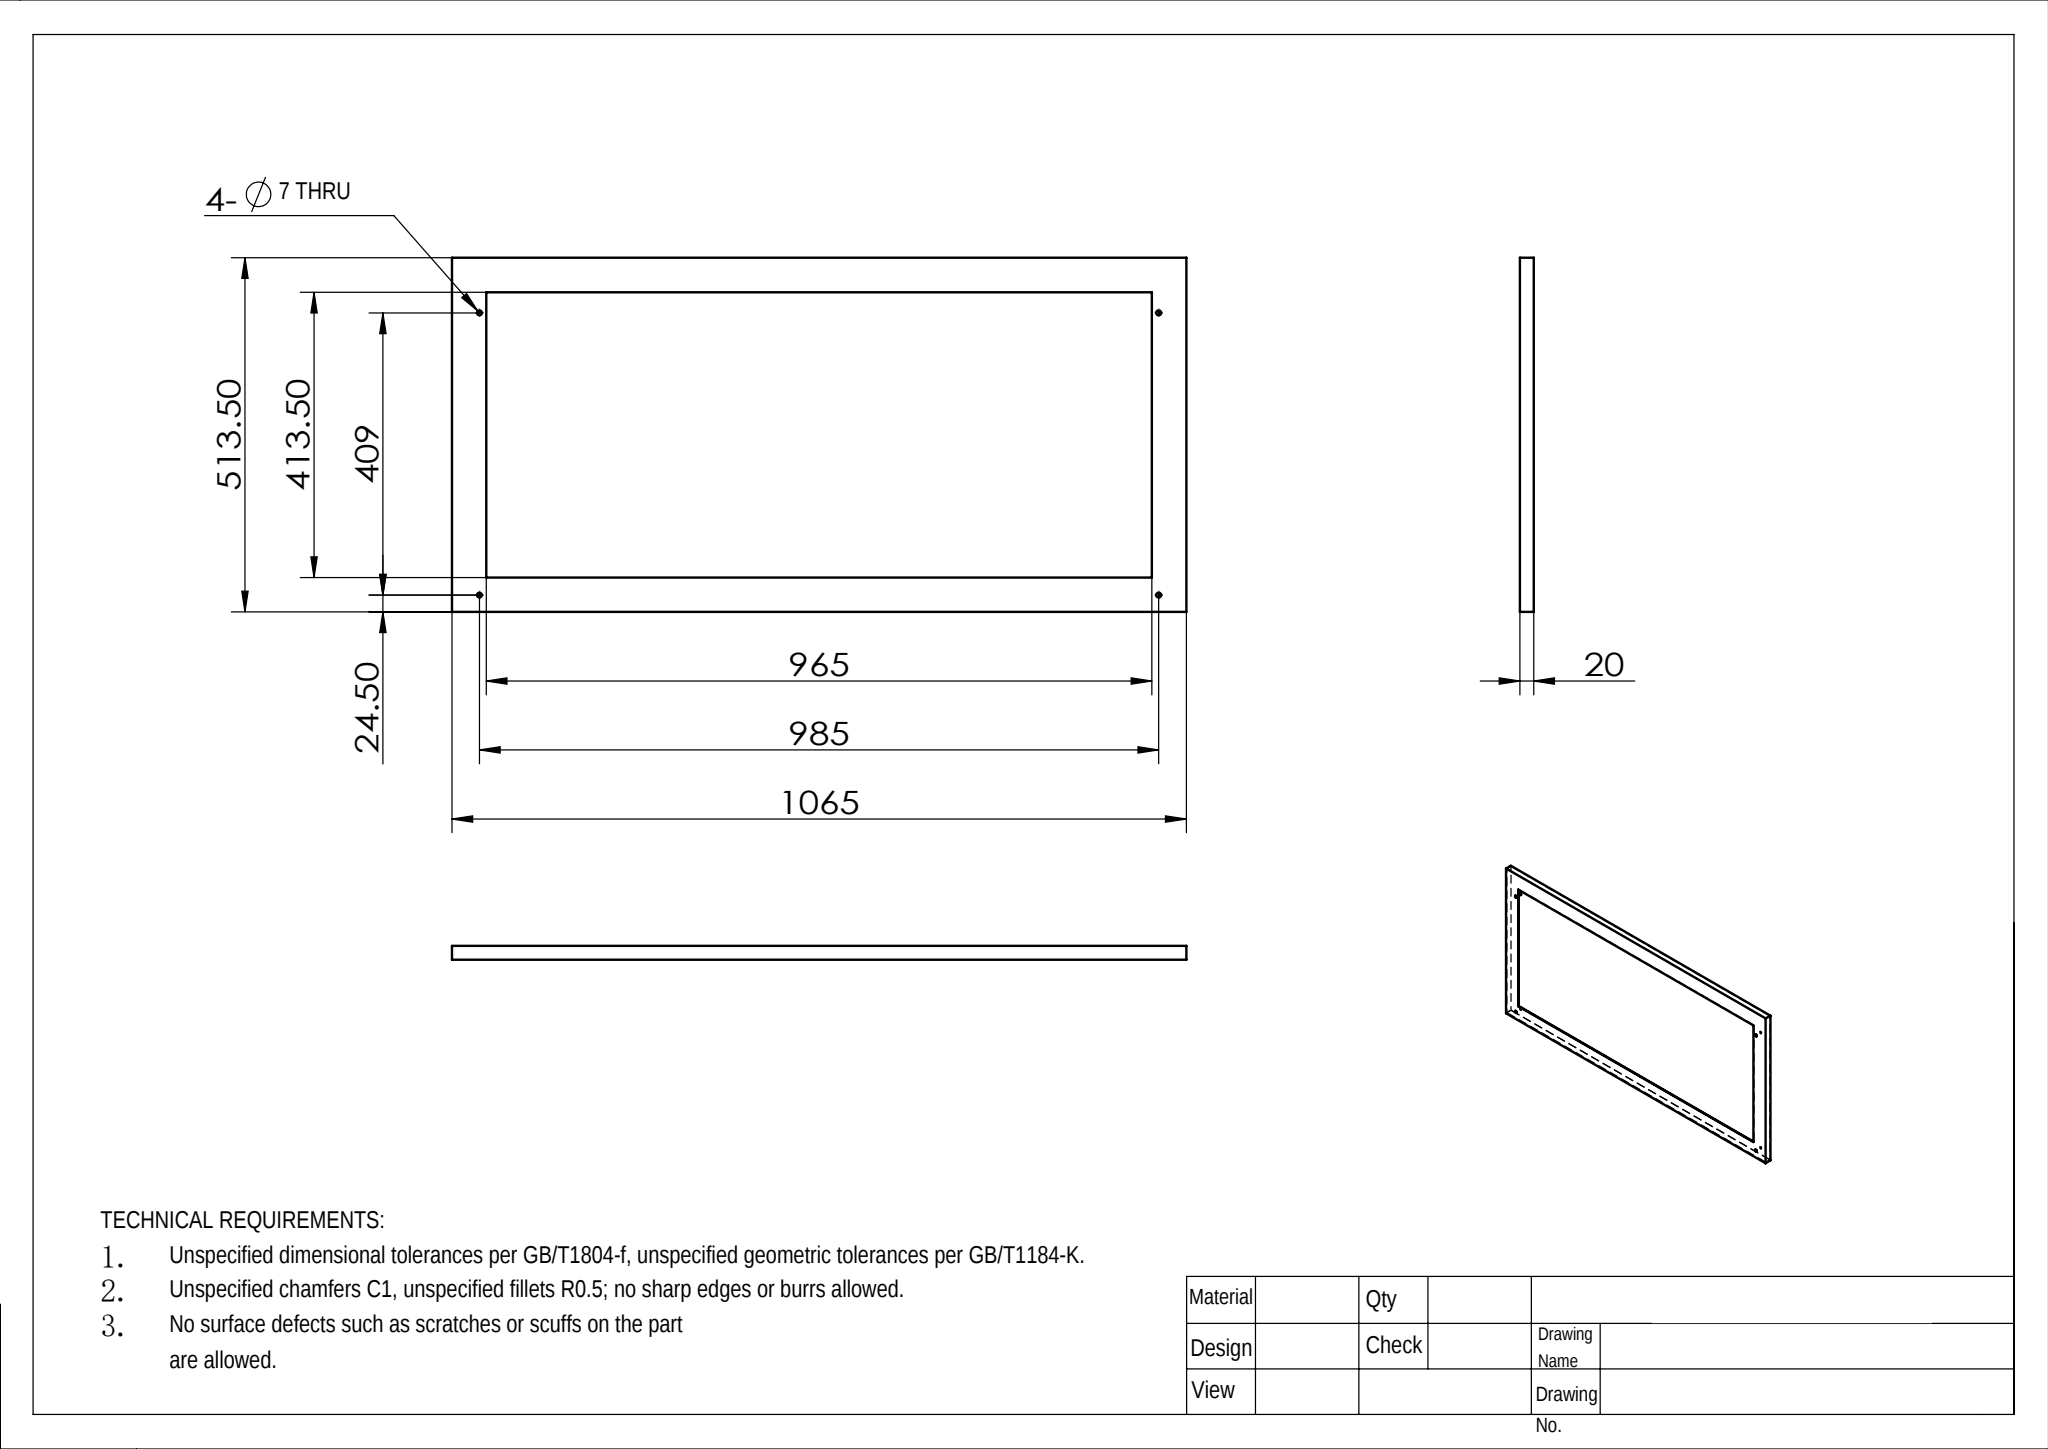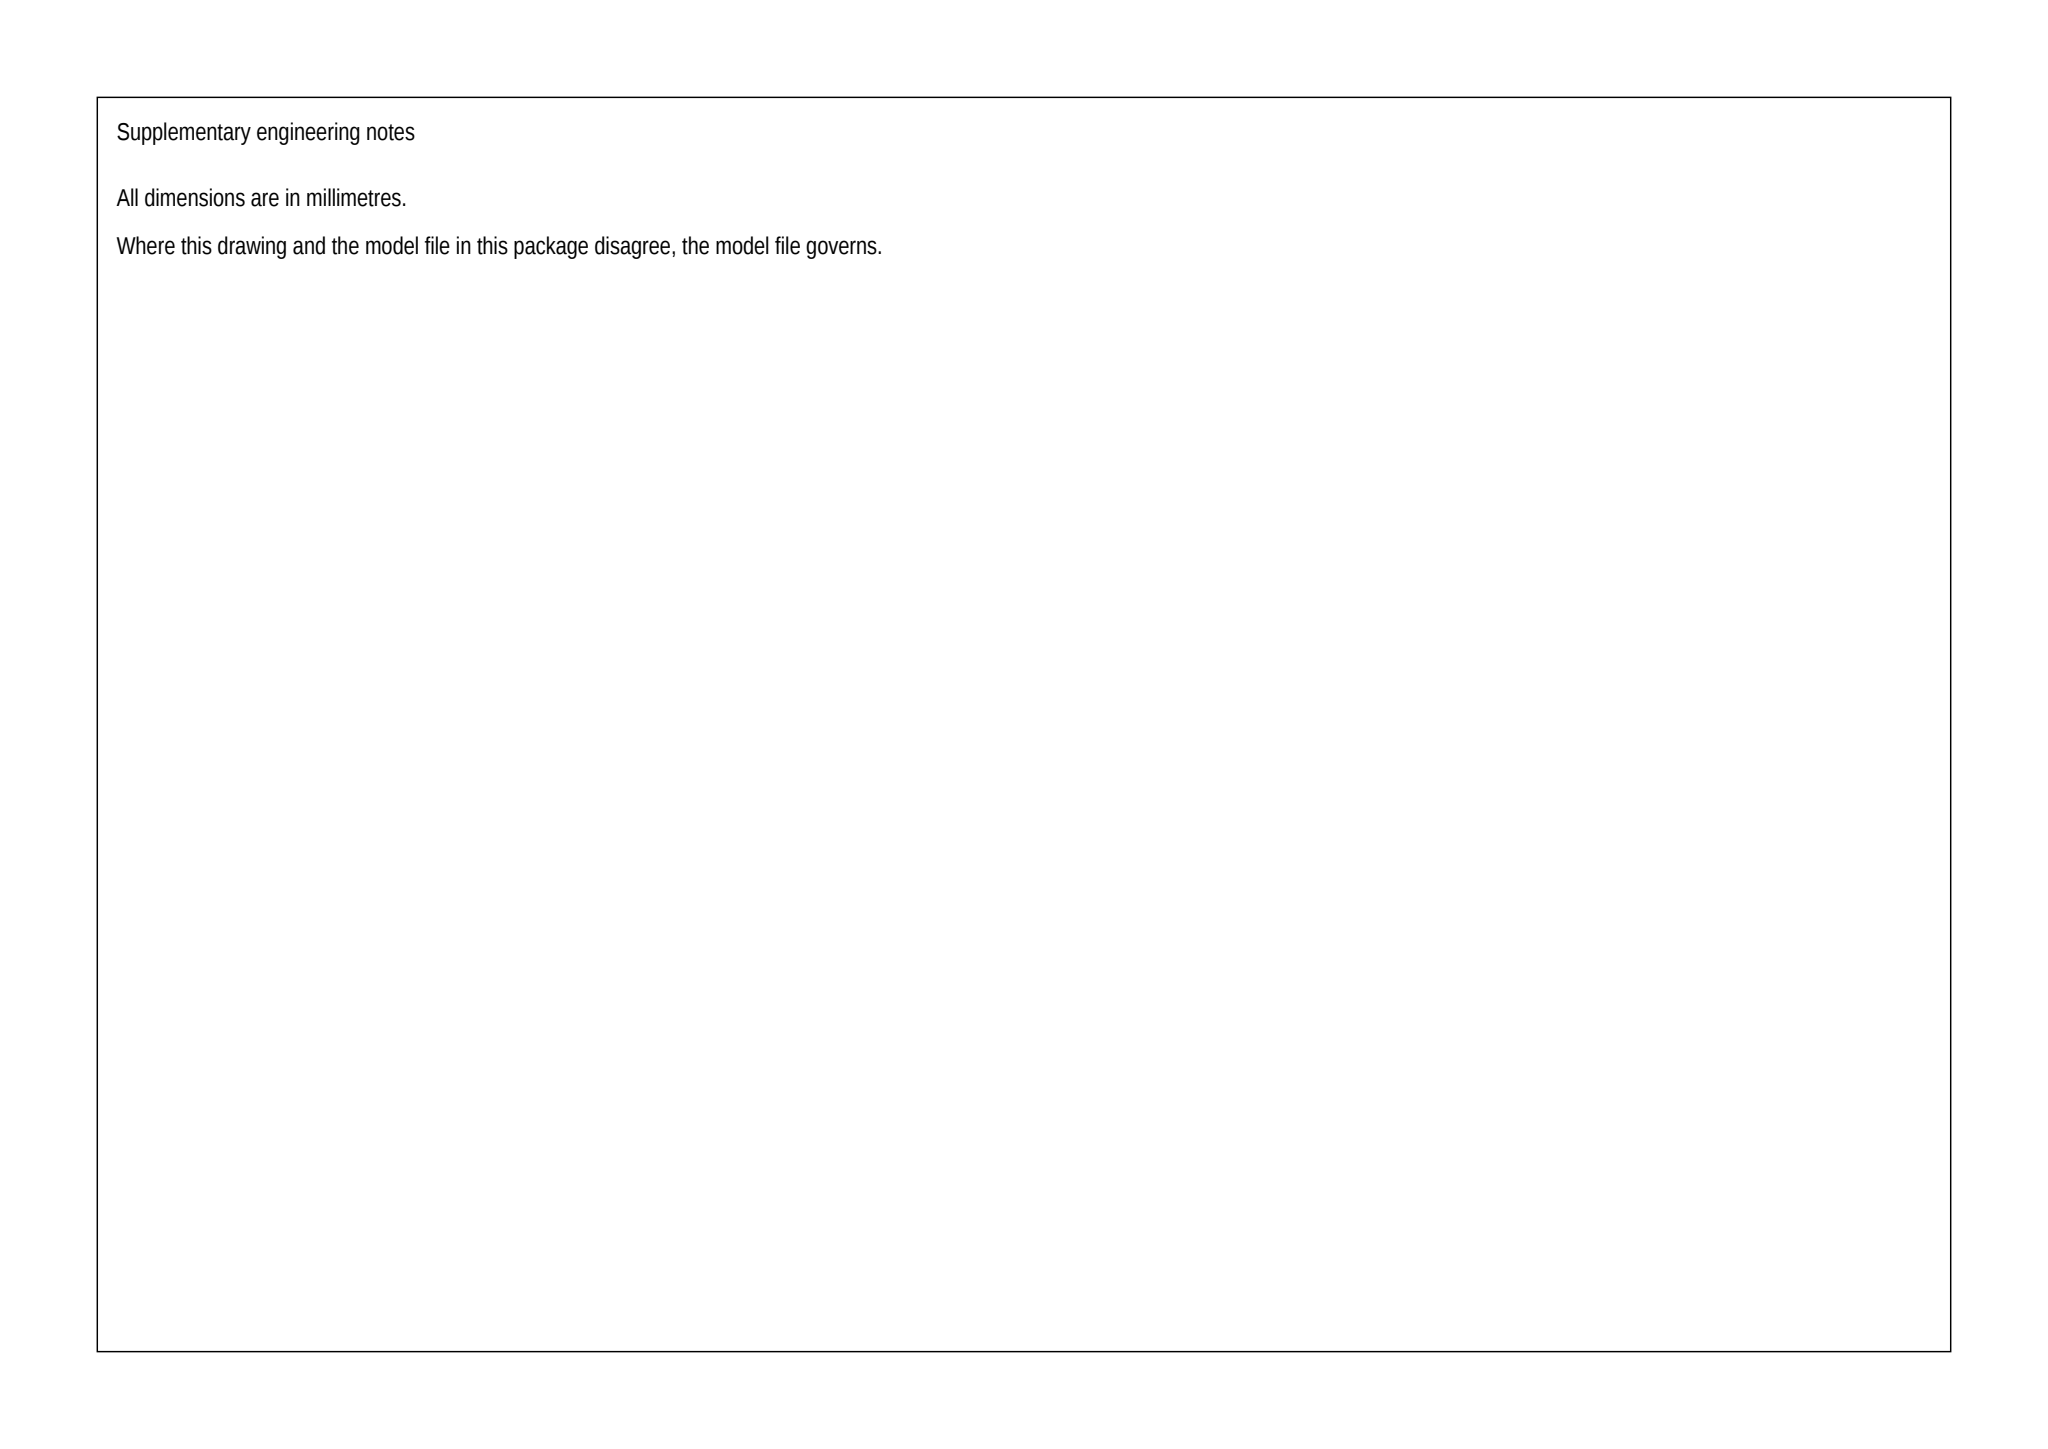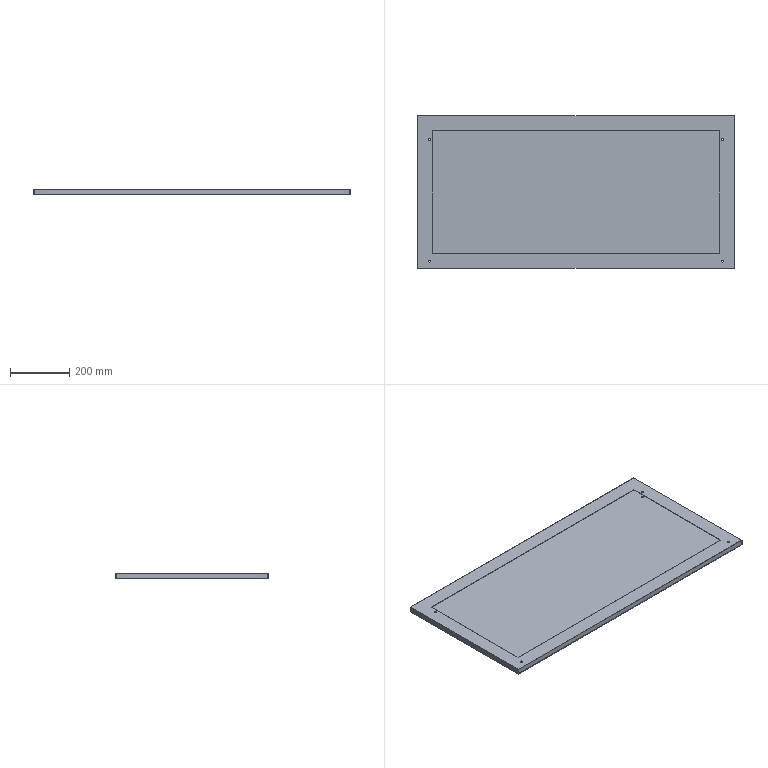Part | SolidWorks | mm | 1 solid | 32 faces | box 1065 x 513.5 x 20 mm | volume 1121980 mm3 | cylinder 16 | plane 16 | commonest cylinder face diameters 7 x16